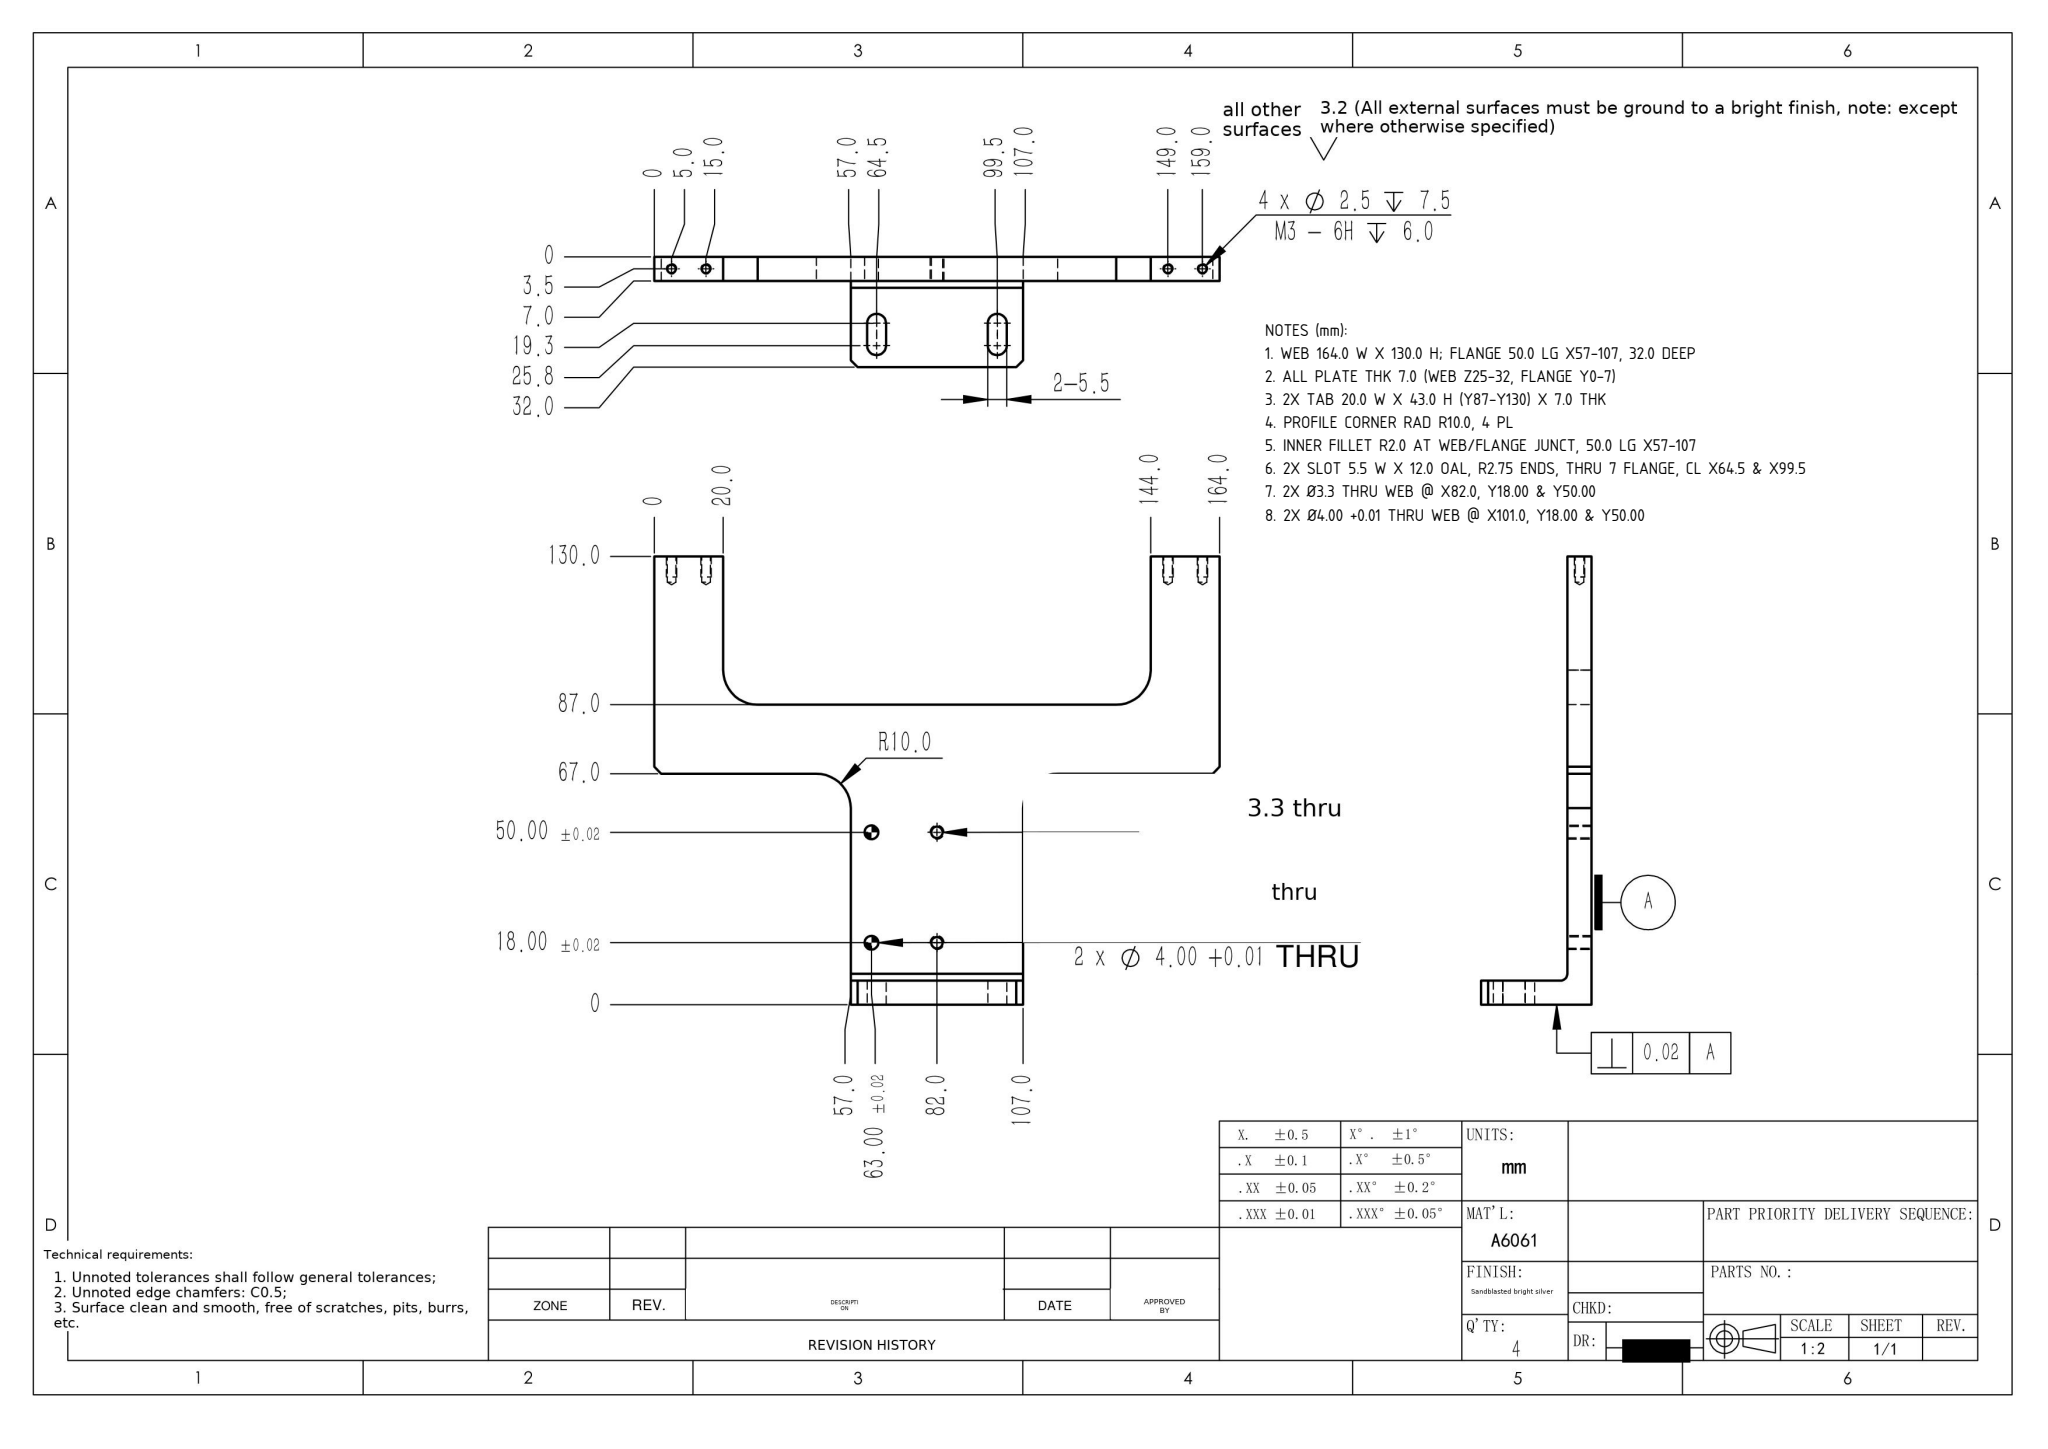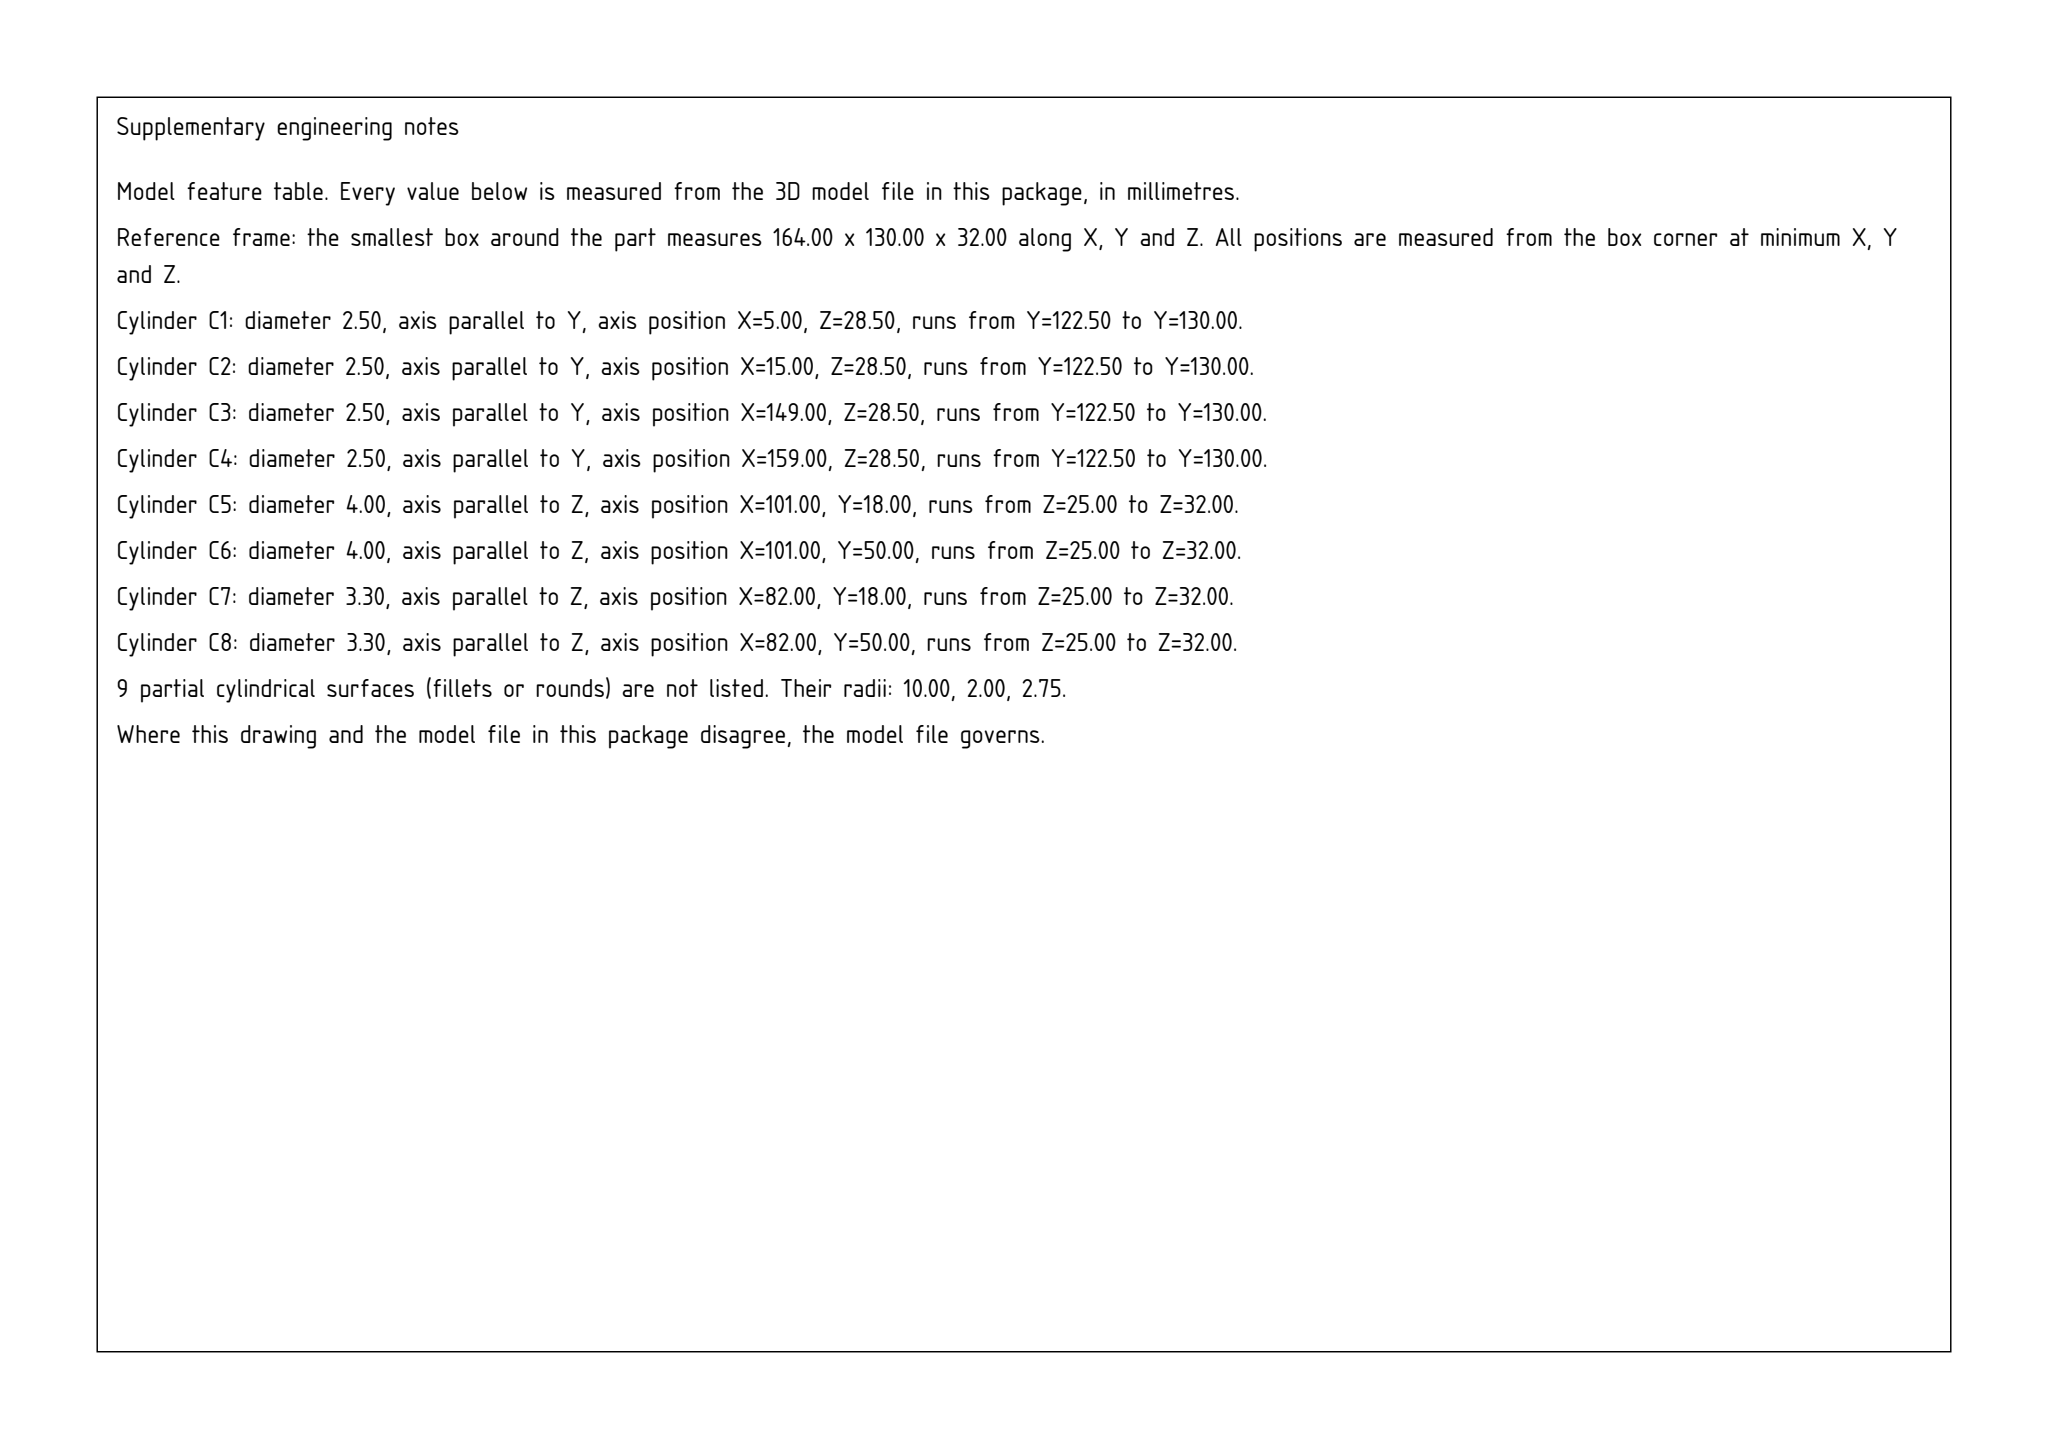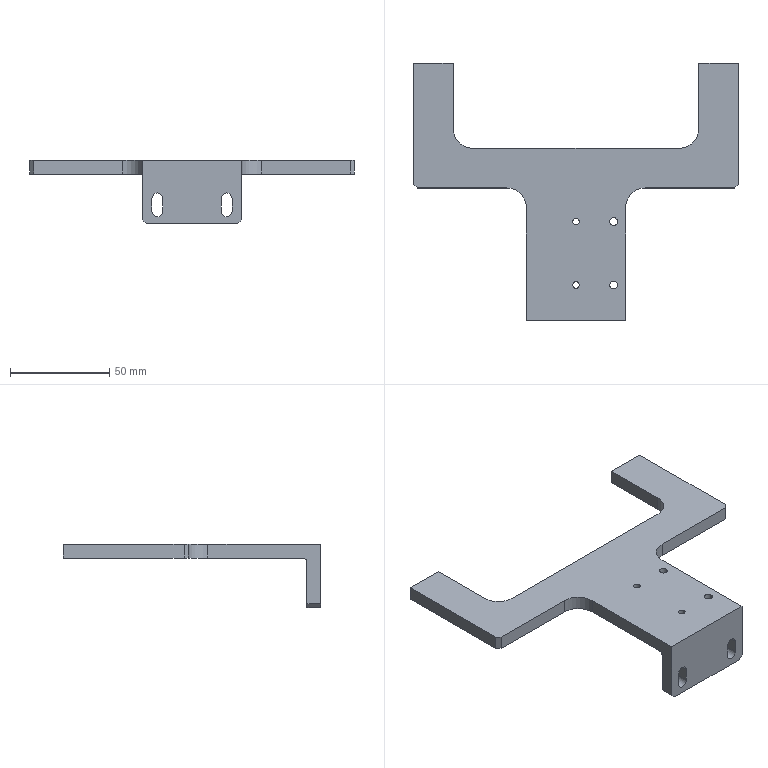Part | SolidWorks | mm | 1 solid | 59 faces | box 164 x 130 x 32 mm | volume 66507 mm3 | cylinder 27 | plane 24 | cone 8 | commonest cylinder face diameters 2.5 x8 5.5 x6 4 x5 3.3 x4 20 x4
Drawing notes:
WEB 164.0 W X 130.0 H; FLANGE 50.0 LG X57-107, 32.0 DEEP | from the solid: bbox 164x130x32; x planes 57.0 and 107.0 bound flange; z planes 0-32
ALL PLATE THK 7.0 (WEB Z25-32, FLANGE Y0-7) | from the solid: z planes 25.0 & 32.0; y planes 0.0 & 7.0; all thru-hole lengths 7.0
2X TAB 20.0 W X 43.0 H (Y87-Y130) X 7.0 THK | from the solid: x planes 0/20 and 144/164; y planes 87 and 130; web thk z25-32 = 7.0
PROFILE CORNER RAD R10.0, 4 PL | from the solid: Ø20 z-axis cyls len 7 at (30,97),(134,97),(47,57),(117,57)
INNER FILLET R2.0 AT WEB/FLANGE JUNCT, 50.0 LG X57-107 | from the solid: Ø4.0 cyl, axis x, pos y=9.0 z=23.0, len 50.0; tangent to y=7 and z=25
2X SLOT 5.5 W X 12.0 OAL, R2.75 ENDS, THRU 7 FLANGE, CL X64.5 & X99.5 | from the solid: Ø5.5 y-axis cyls at x=64.5 & 99.5, z=6.25 & 12.75, len 7.0; planes x61.75/67.25, 96.75/102.25; 6.5 ctr-ctr + 5.5 = 12.0
2X Ø3.3 THRU WEB @ X82.0, Y18.00 & Y50.00 | from the solid: Ø3.3 z-axis cyls at (82,18) and (82,50), len 7 = web thk
2X Ø4.00 +0.01 THRU WEB @ X101.0, Y18.00 & Y50.00 | from the solid: Ø4.0 z-axis cyls at (101,18) and (101,50), len 7 thru web